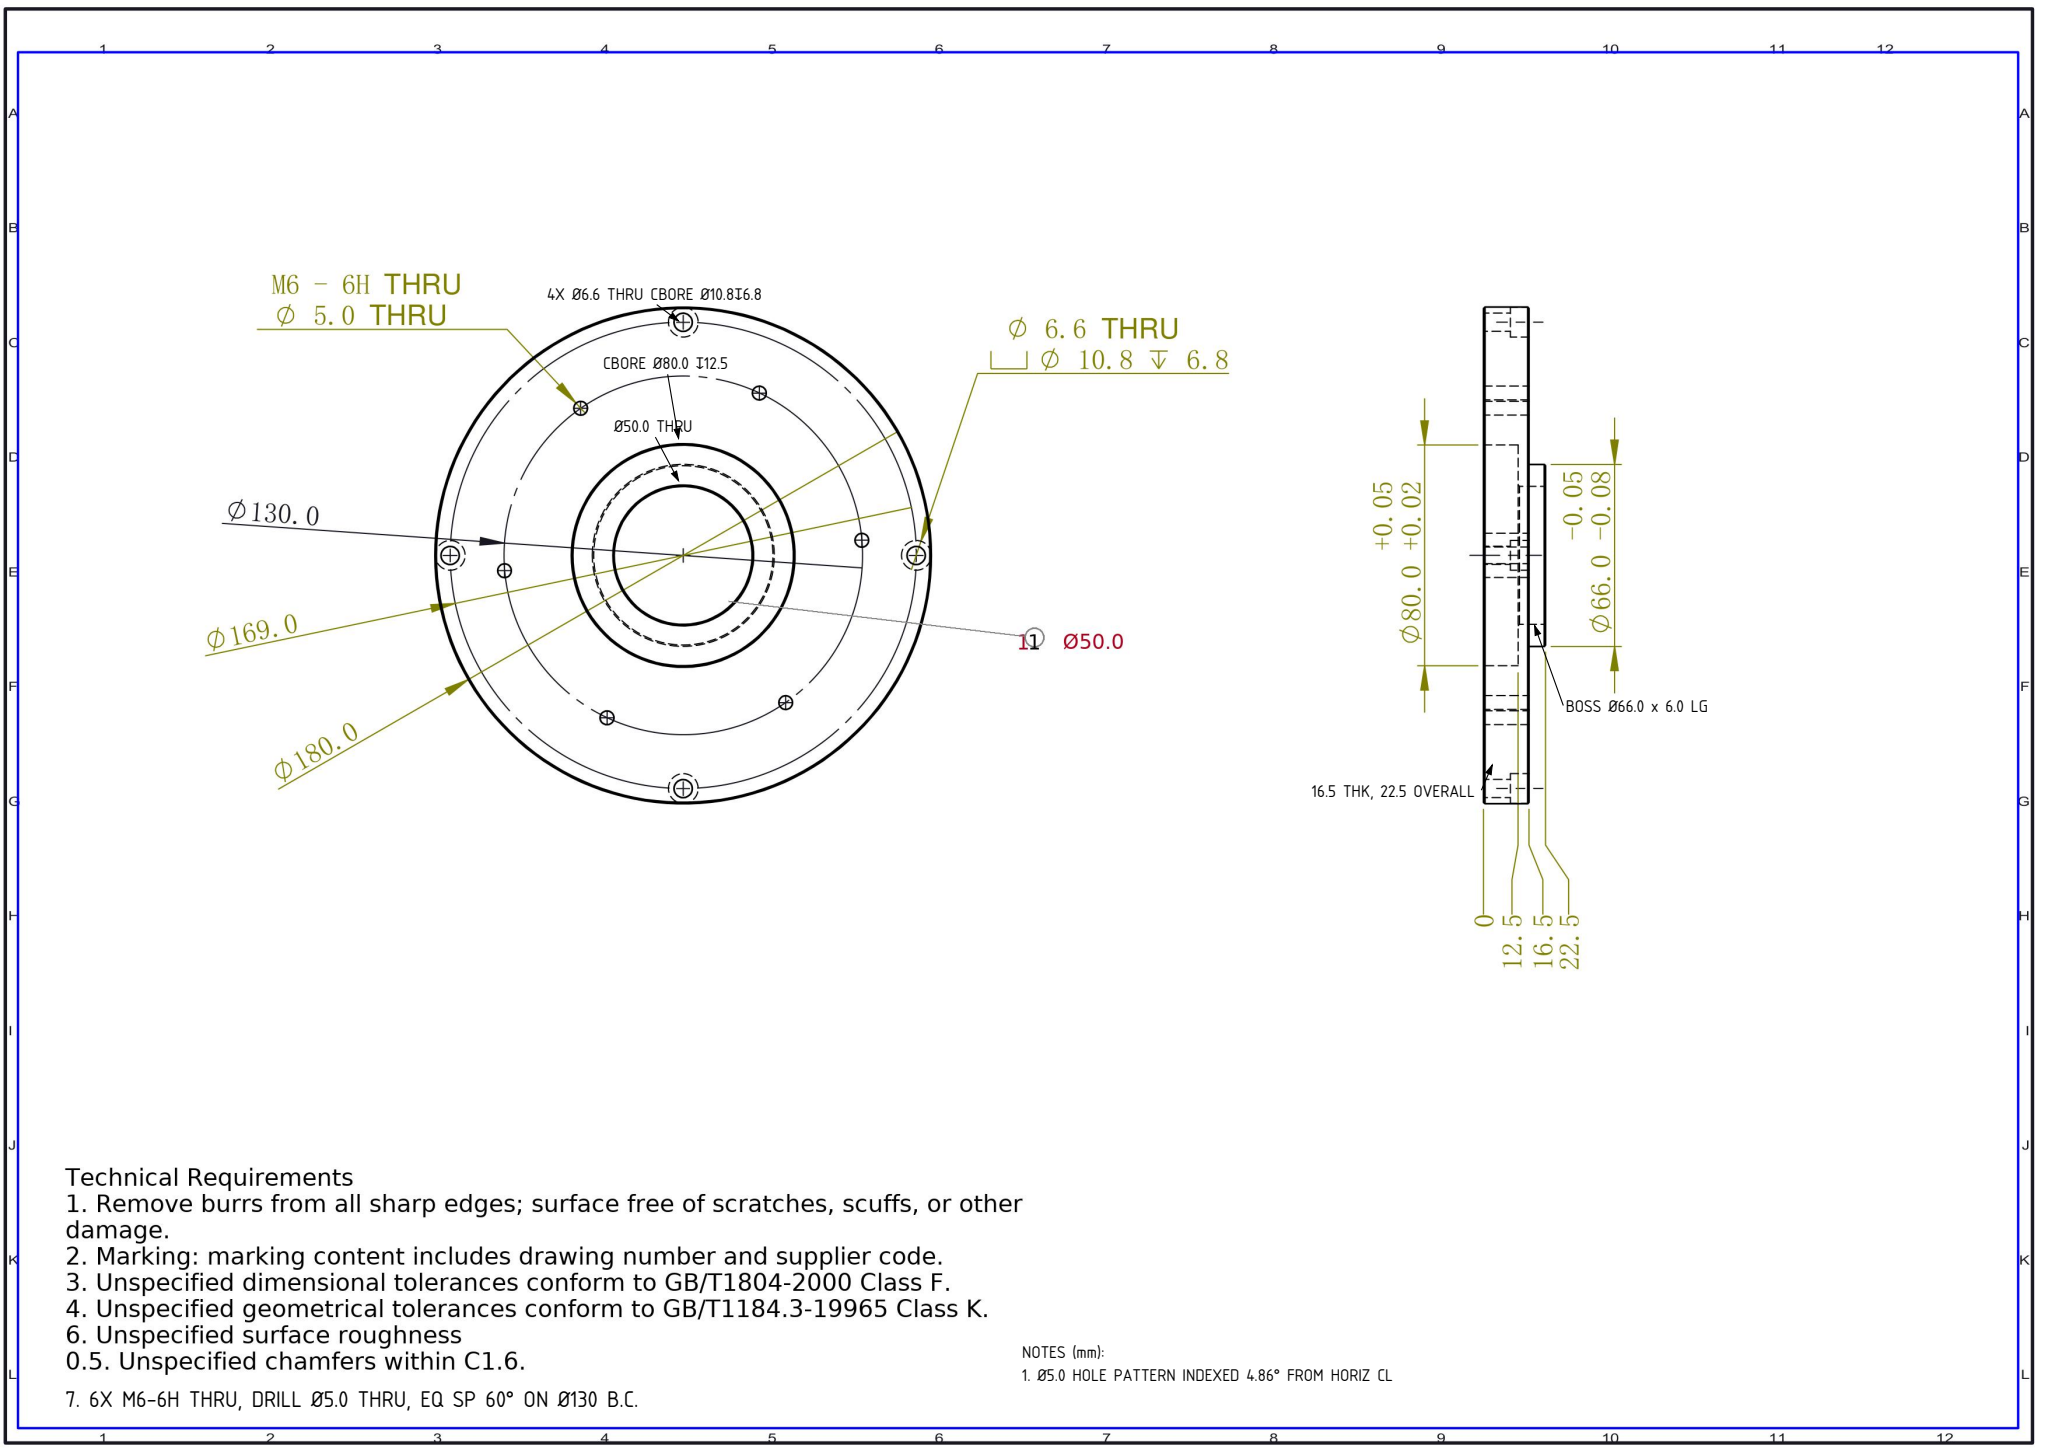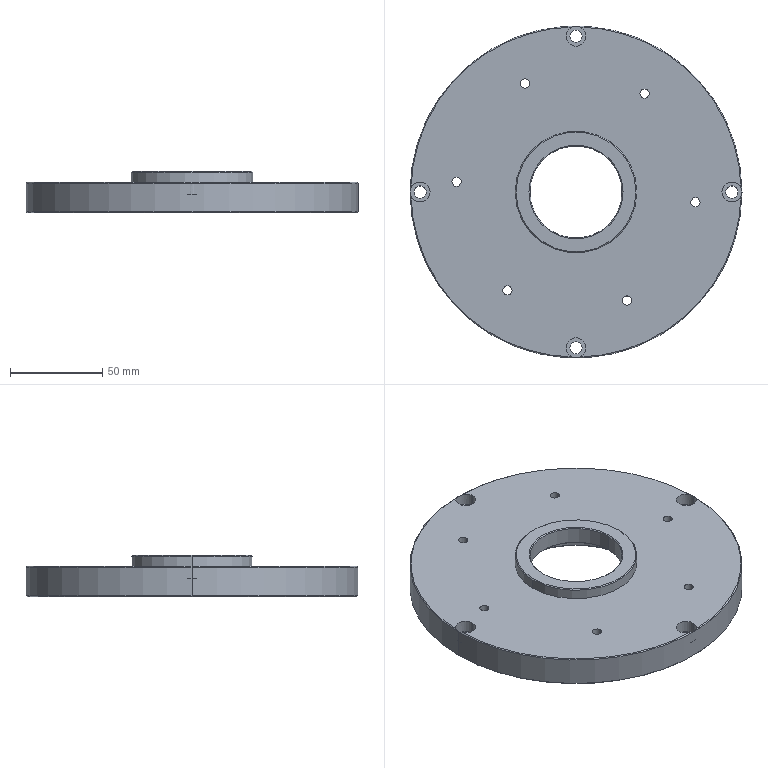Part | SolidWorks | mm | 1 solid | 56 faces | box 180 x 180 x 22.5 mm | volume 351934 mm3 | cylinder 36 | cone 12 | plane 8 | commonest cylinder face diameters 5 x12 10.8 x8 6.6 x8 66 x2 50 x2 180 x2 80 x2
Drawing notes:
PLATE Ø180.0 x 16.5 THK; OVERALL THK 22.5 INCL BOSS | from the solid: Ø180 cyl L15.5 + 0.5 chamfers = 16.5; bbox z = 22.5
CTR BORE Ø50.0 THRU | from the solid: Ø50 cyl L9.0 on axis (90,90), breaks thru to z=22.5
CBORE Ø80.0 +0.05/+0.02 DP 12.5 FROM BACK FACE | from the solid: Ø80 cyl L12.0 from z=0, step plane at z=12.5
BOSS Ø66.0 -0.05/-0.08 x 6.0 LG, FROM 16.5 FACE TO 22.5 | from the solid: Ø66 cyl L5.5 (+0.5 chamfer) between planes z=16.5 and z=22.5
6X M6-6H THRU, DRILL Ø5.0 THRU, EQ SP 60° ON Ø130 B.C. | from the solid: Six Ø5.0 z-cyl L16.5 at R65.0 from ctr (90,90), 60° spacing
Ø5.0 HOLE PATTERN INDEXED 4.86° FROM HORIZ CL | from the solid: Hole (154.77,84.49): dx=64.77, dy=-5.51 -> -4.86° from +X CL
4X Ø6.6 THRU, CBORE Ø10.8 DP 6.8, EQ SP 90° ON Ø169 B.C. | from the solid: Ø6.6 L9.7 + Ø10.8 L6.8 at (5.5,90),(90,5.5),(90,174.5),(174.5,90) = R84.5